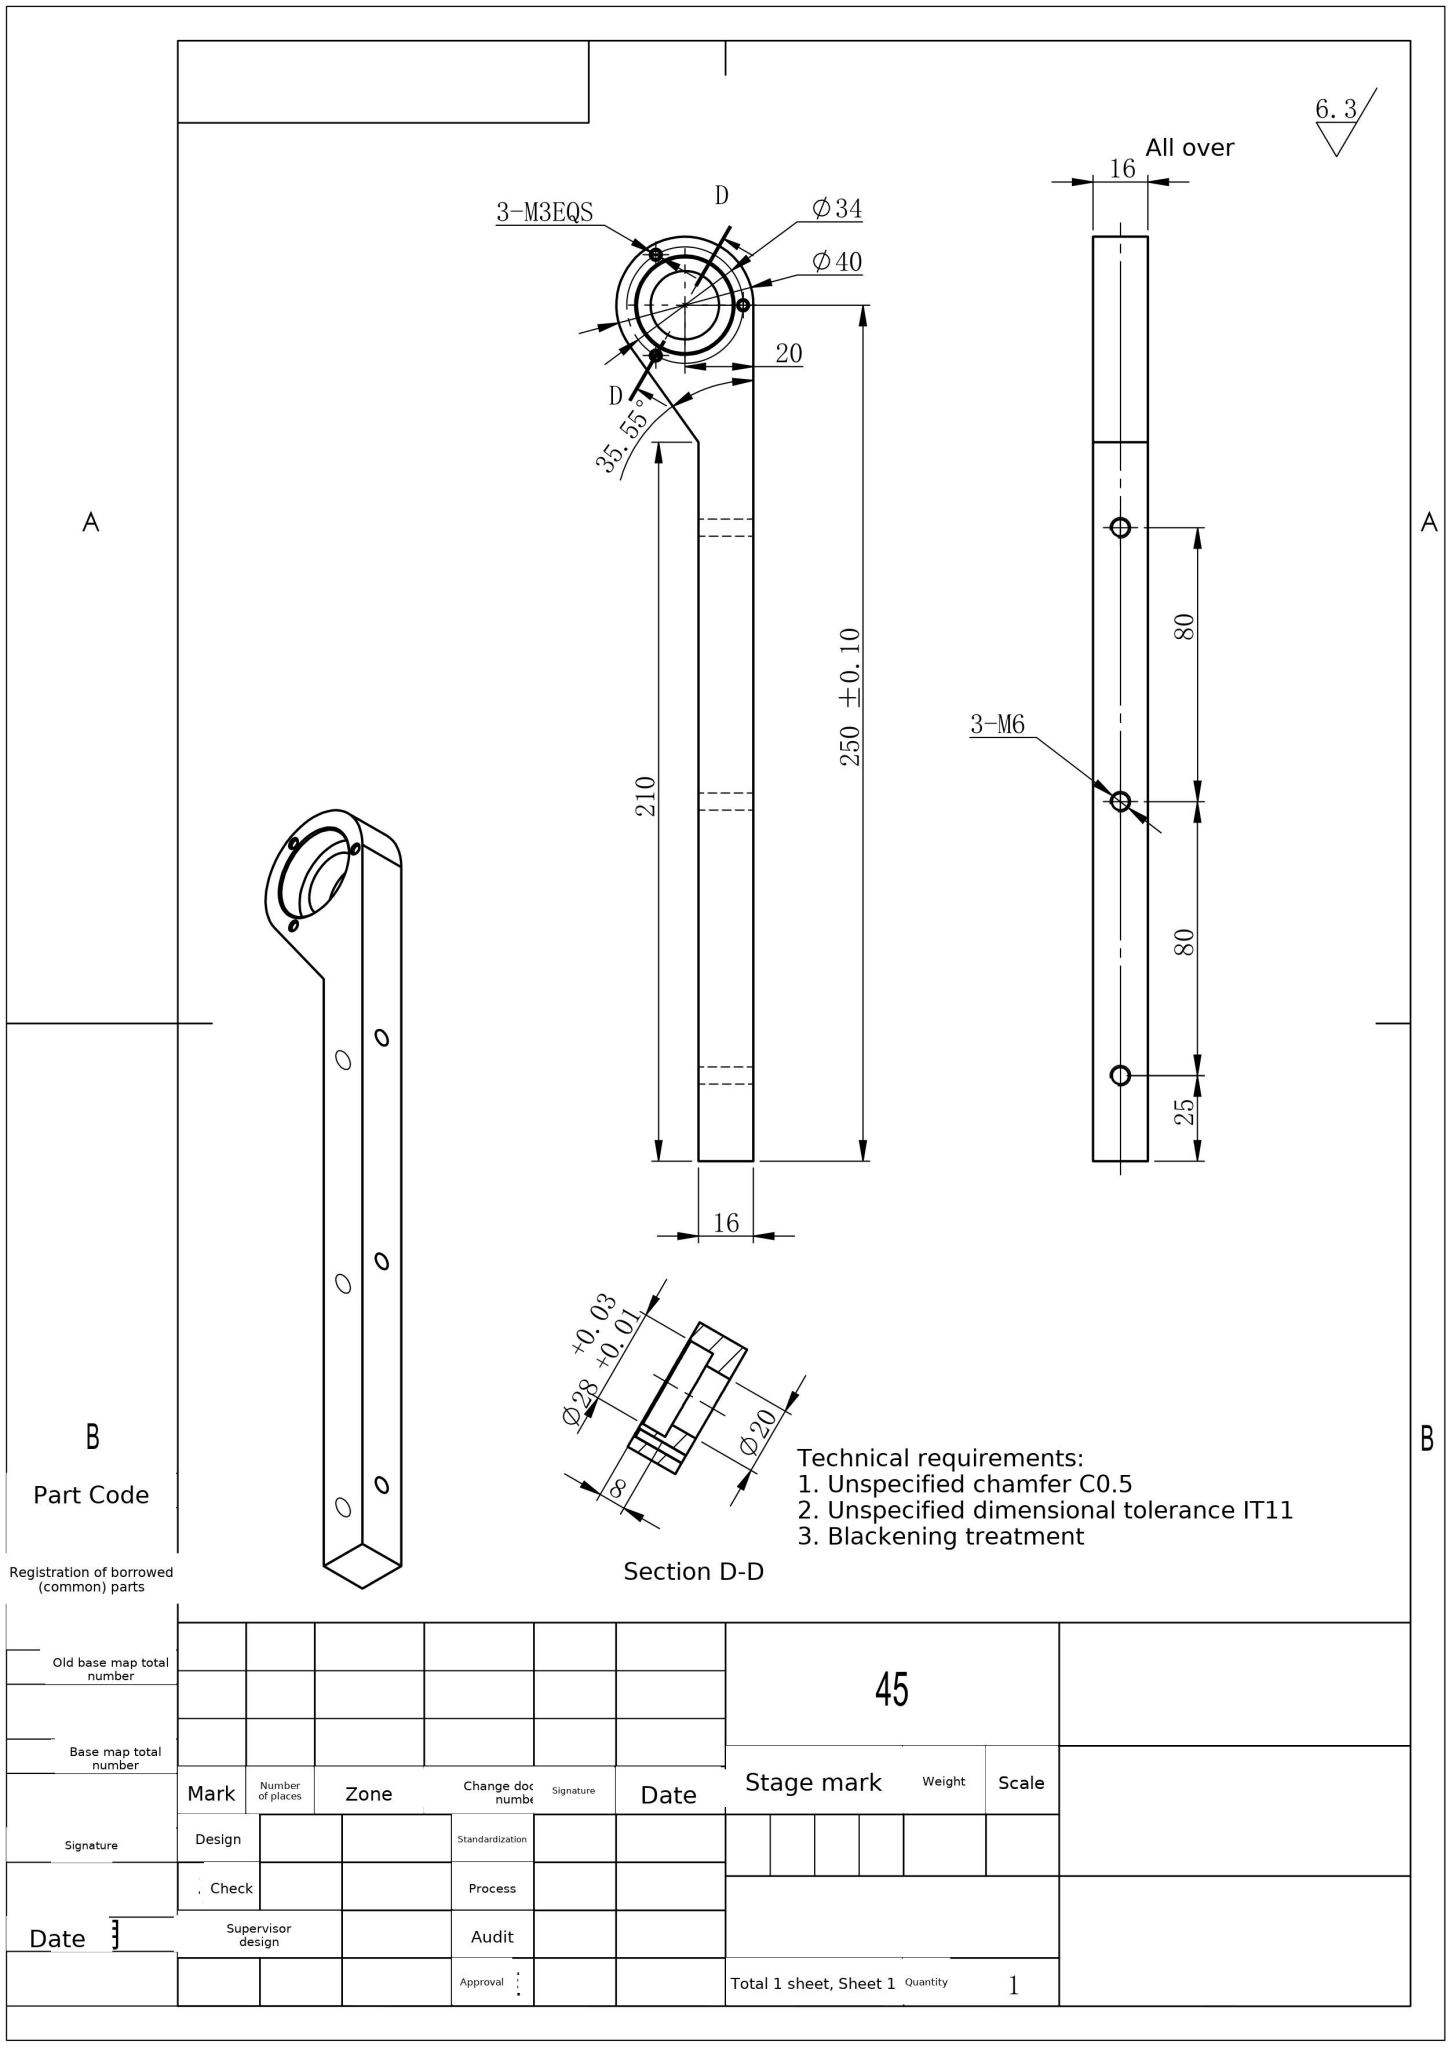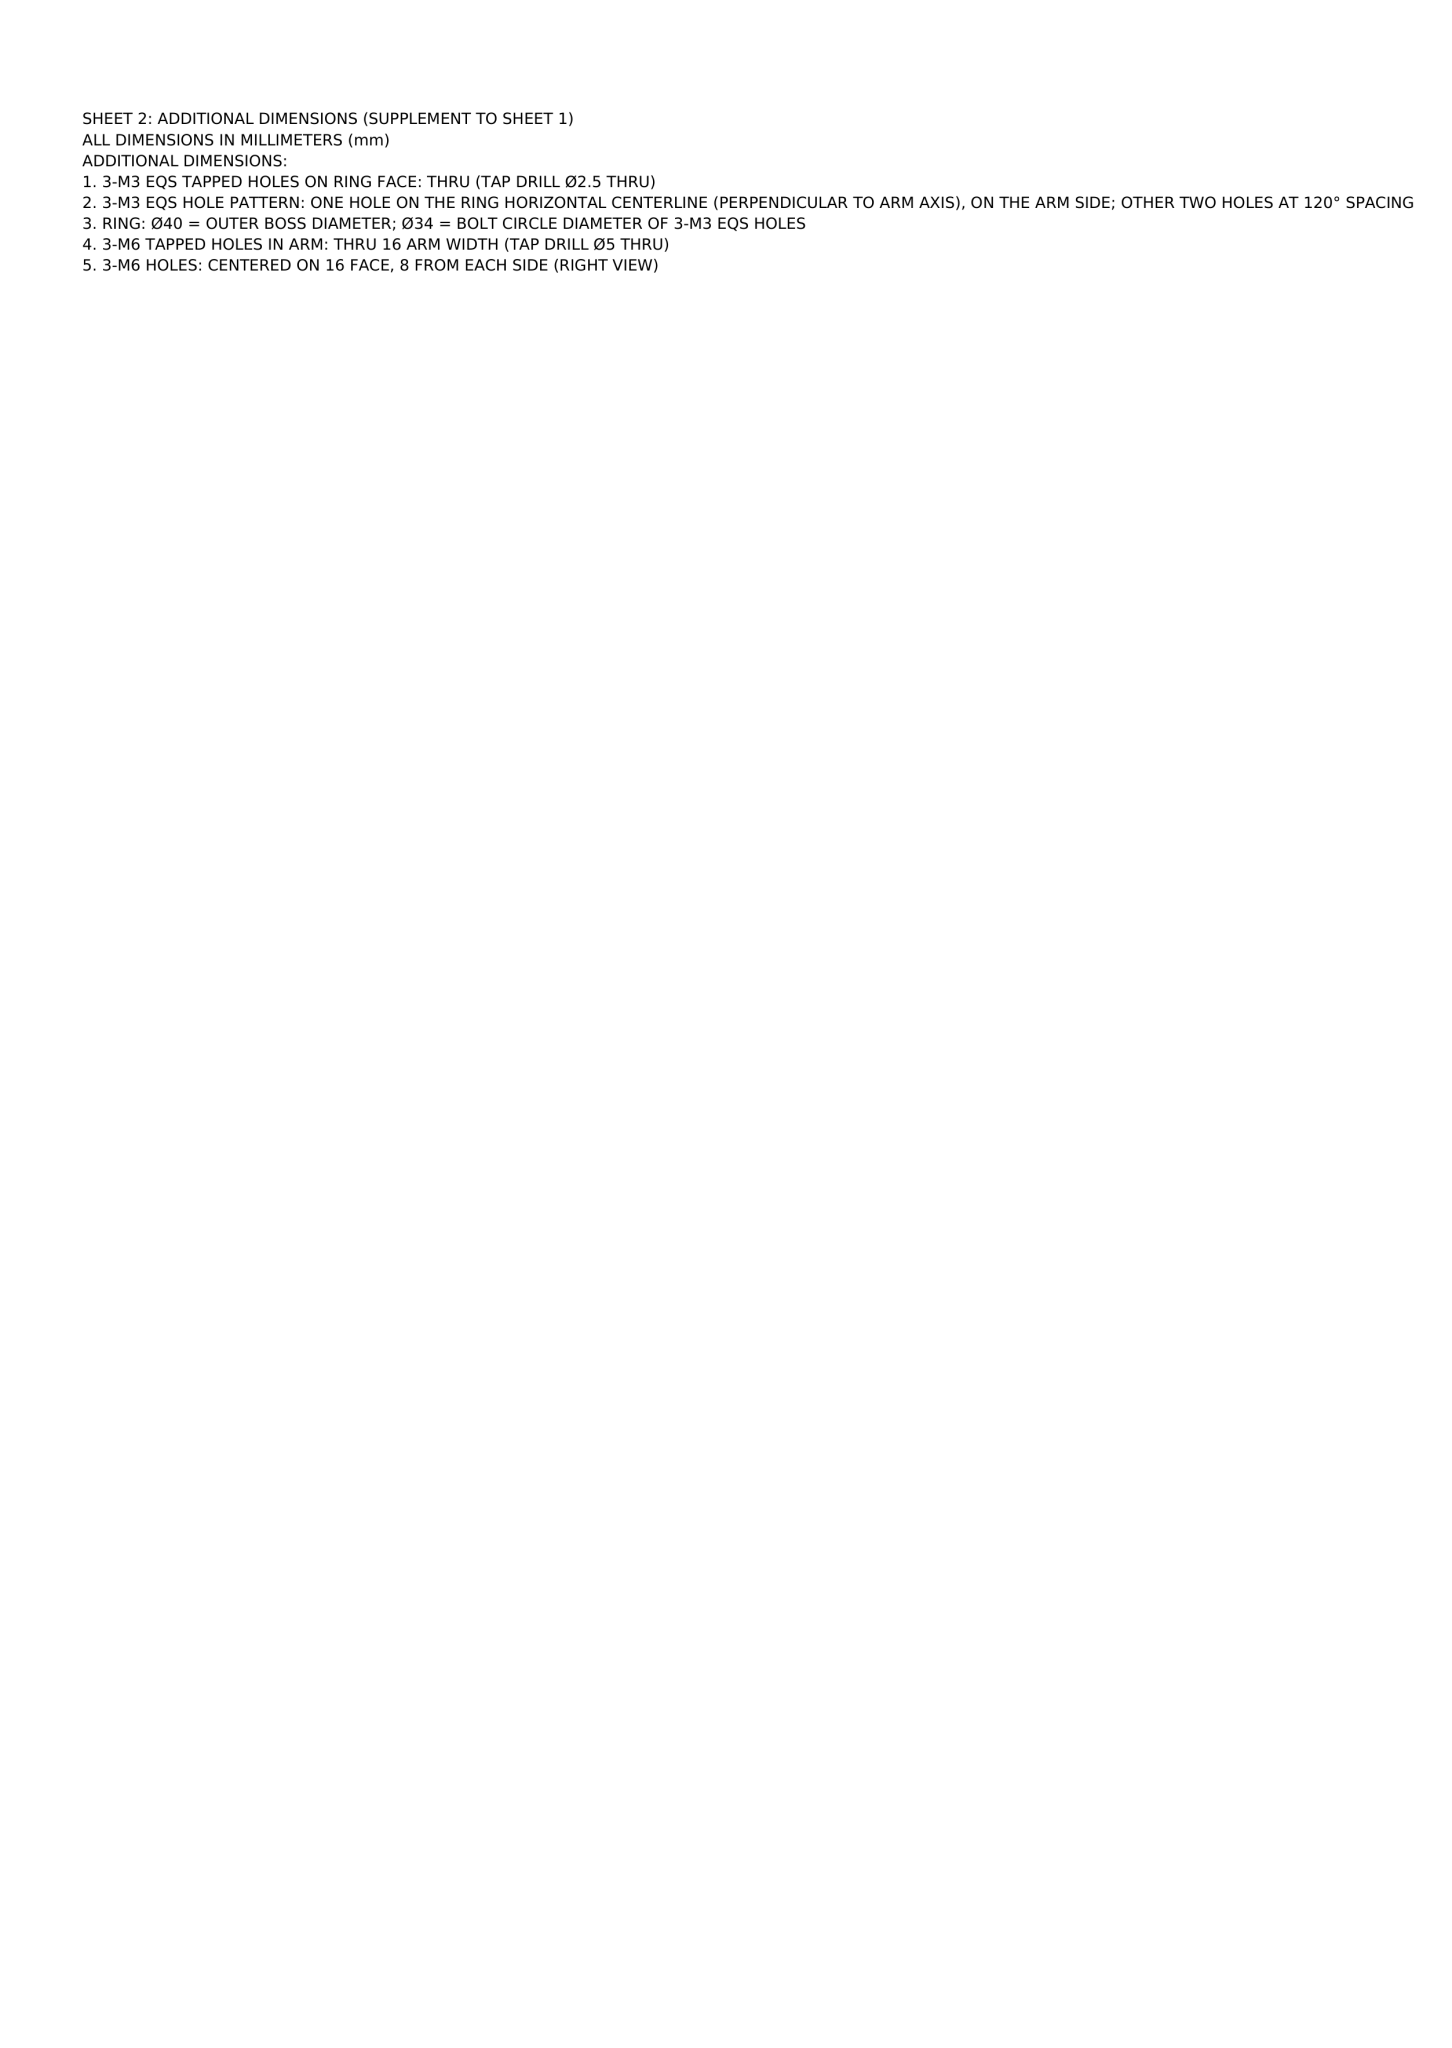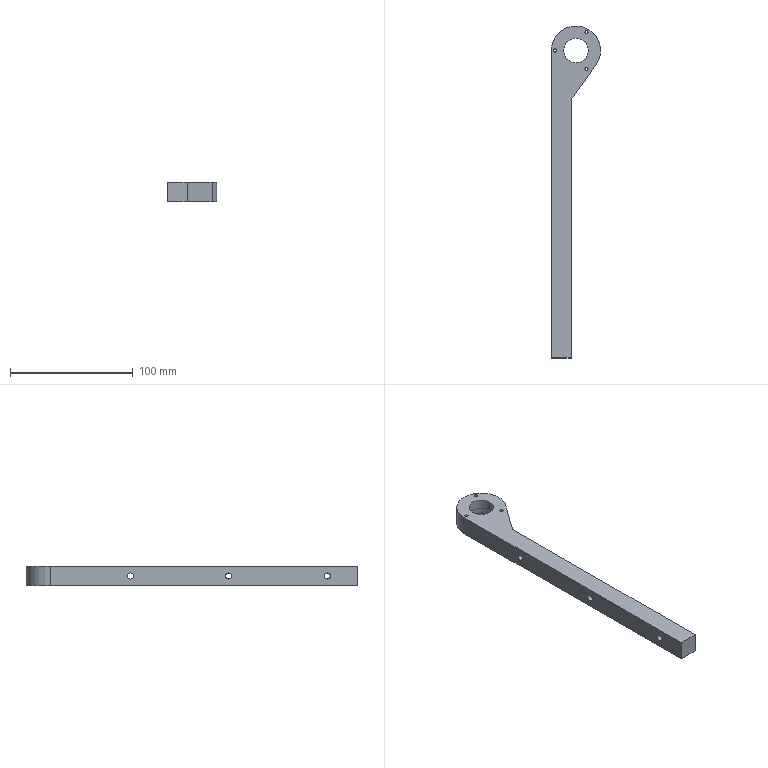Part | NX | mm | 1 solid | 32 faces | box 40 x 270 x 16 mm | volume 74266 mm3 | cylinder 17 | cone 8 | plane 7 | commonest cylinder face diameters 5 x6 2.5 x6 20 x2 28 x2 40 x1